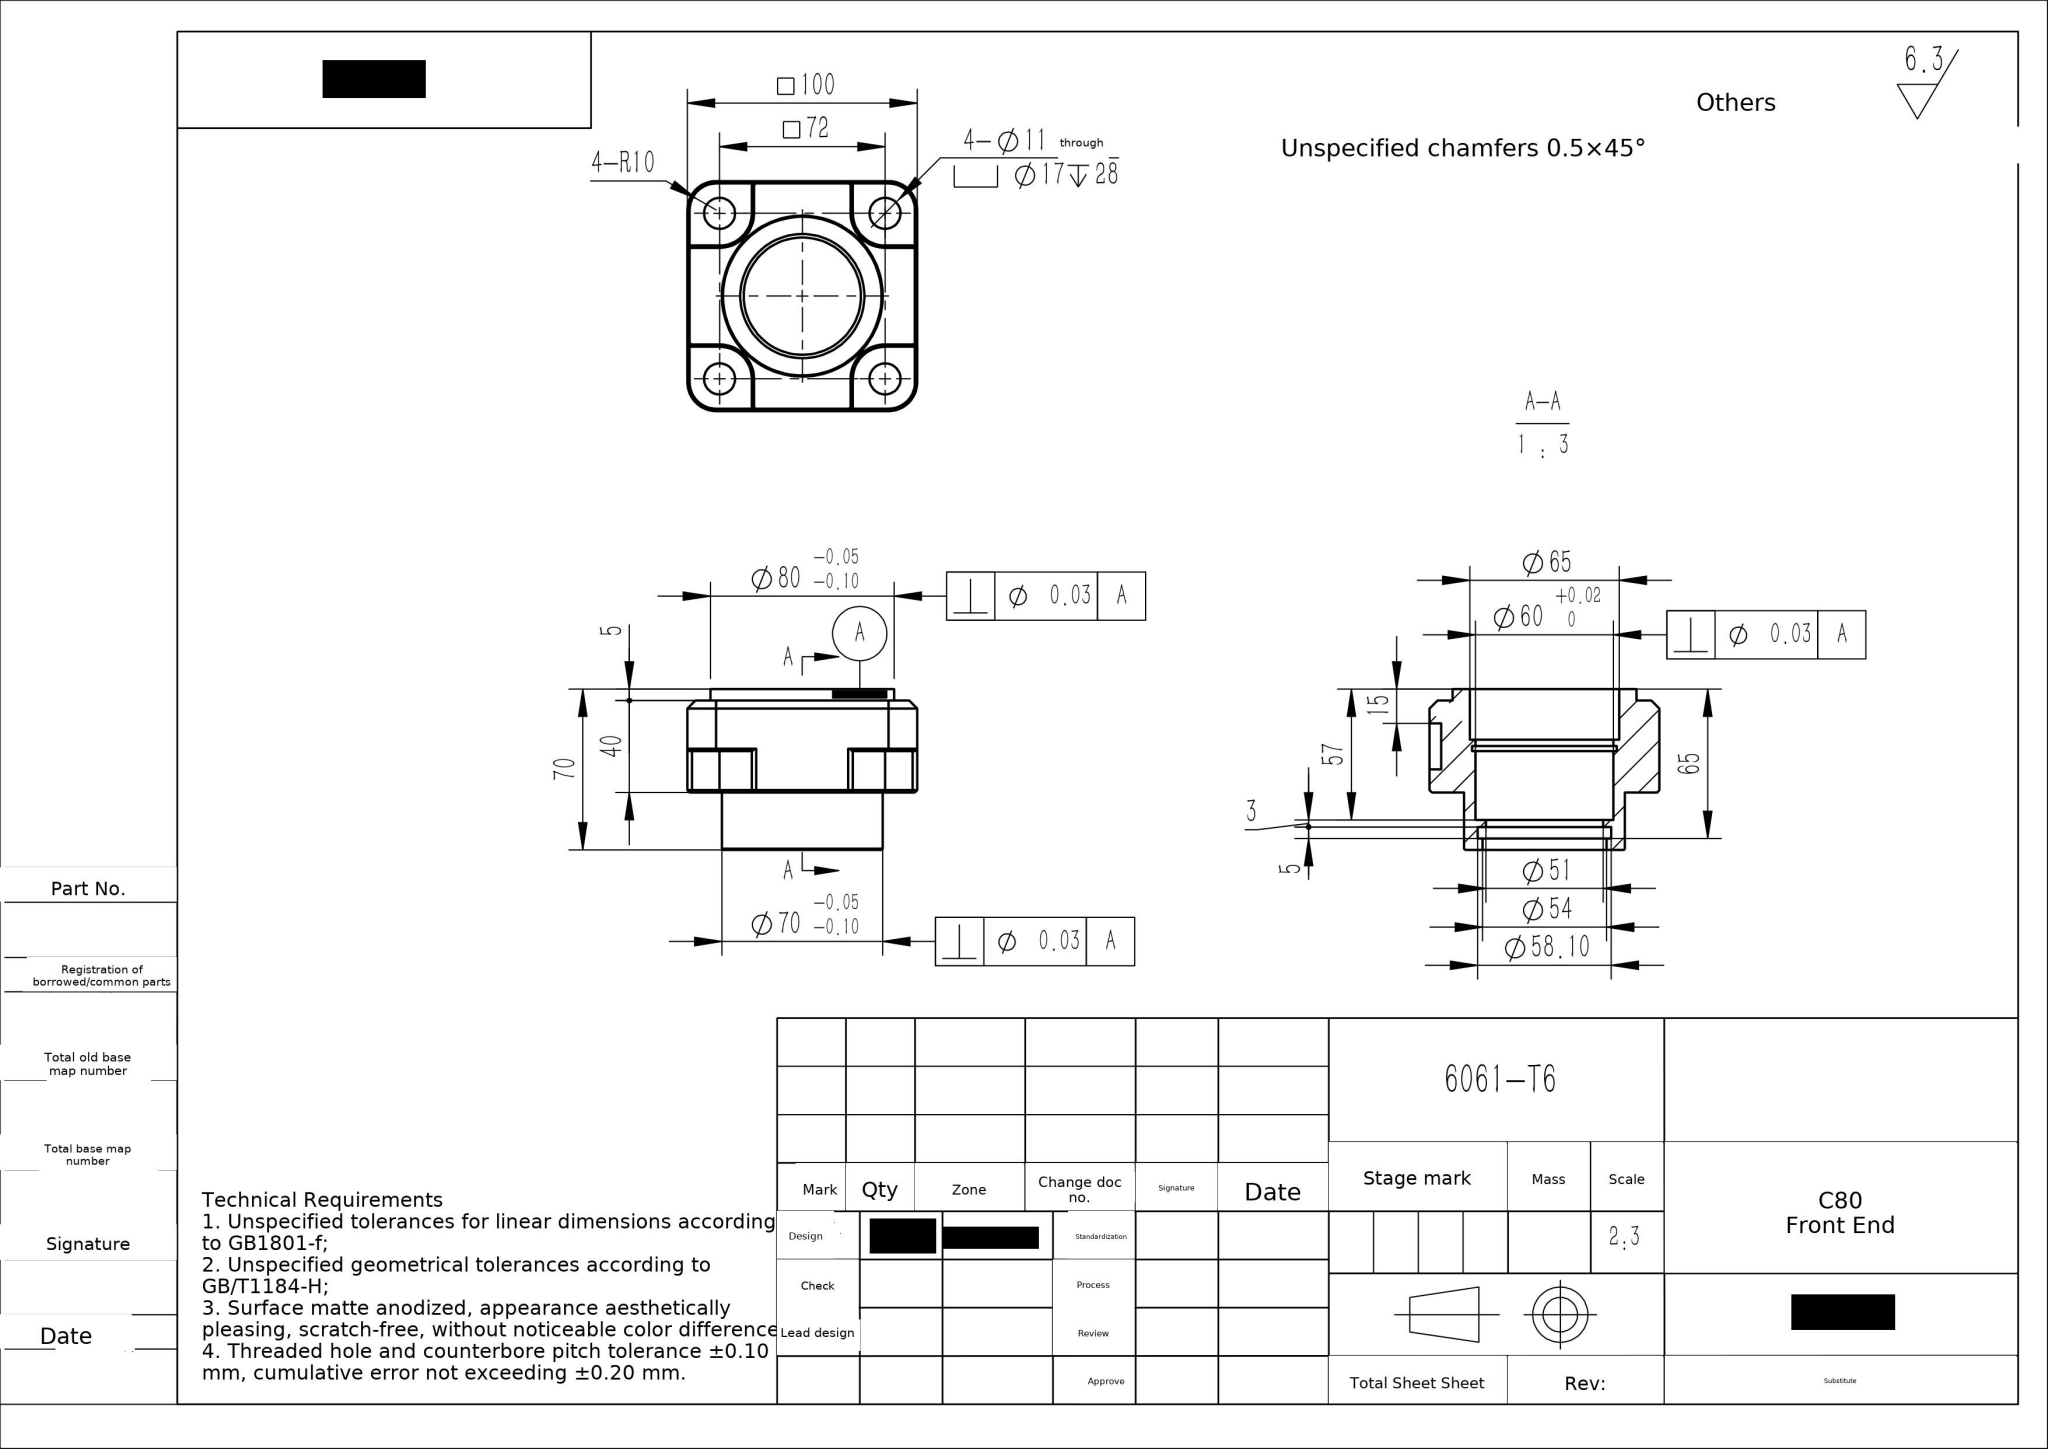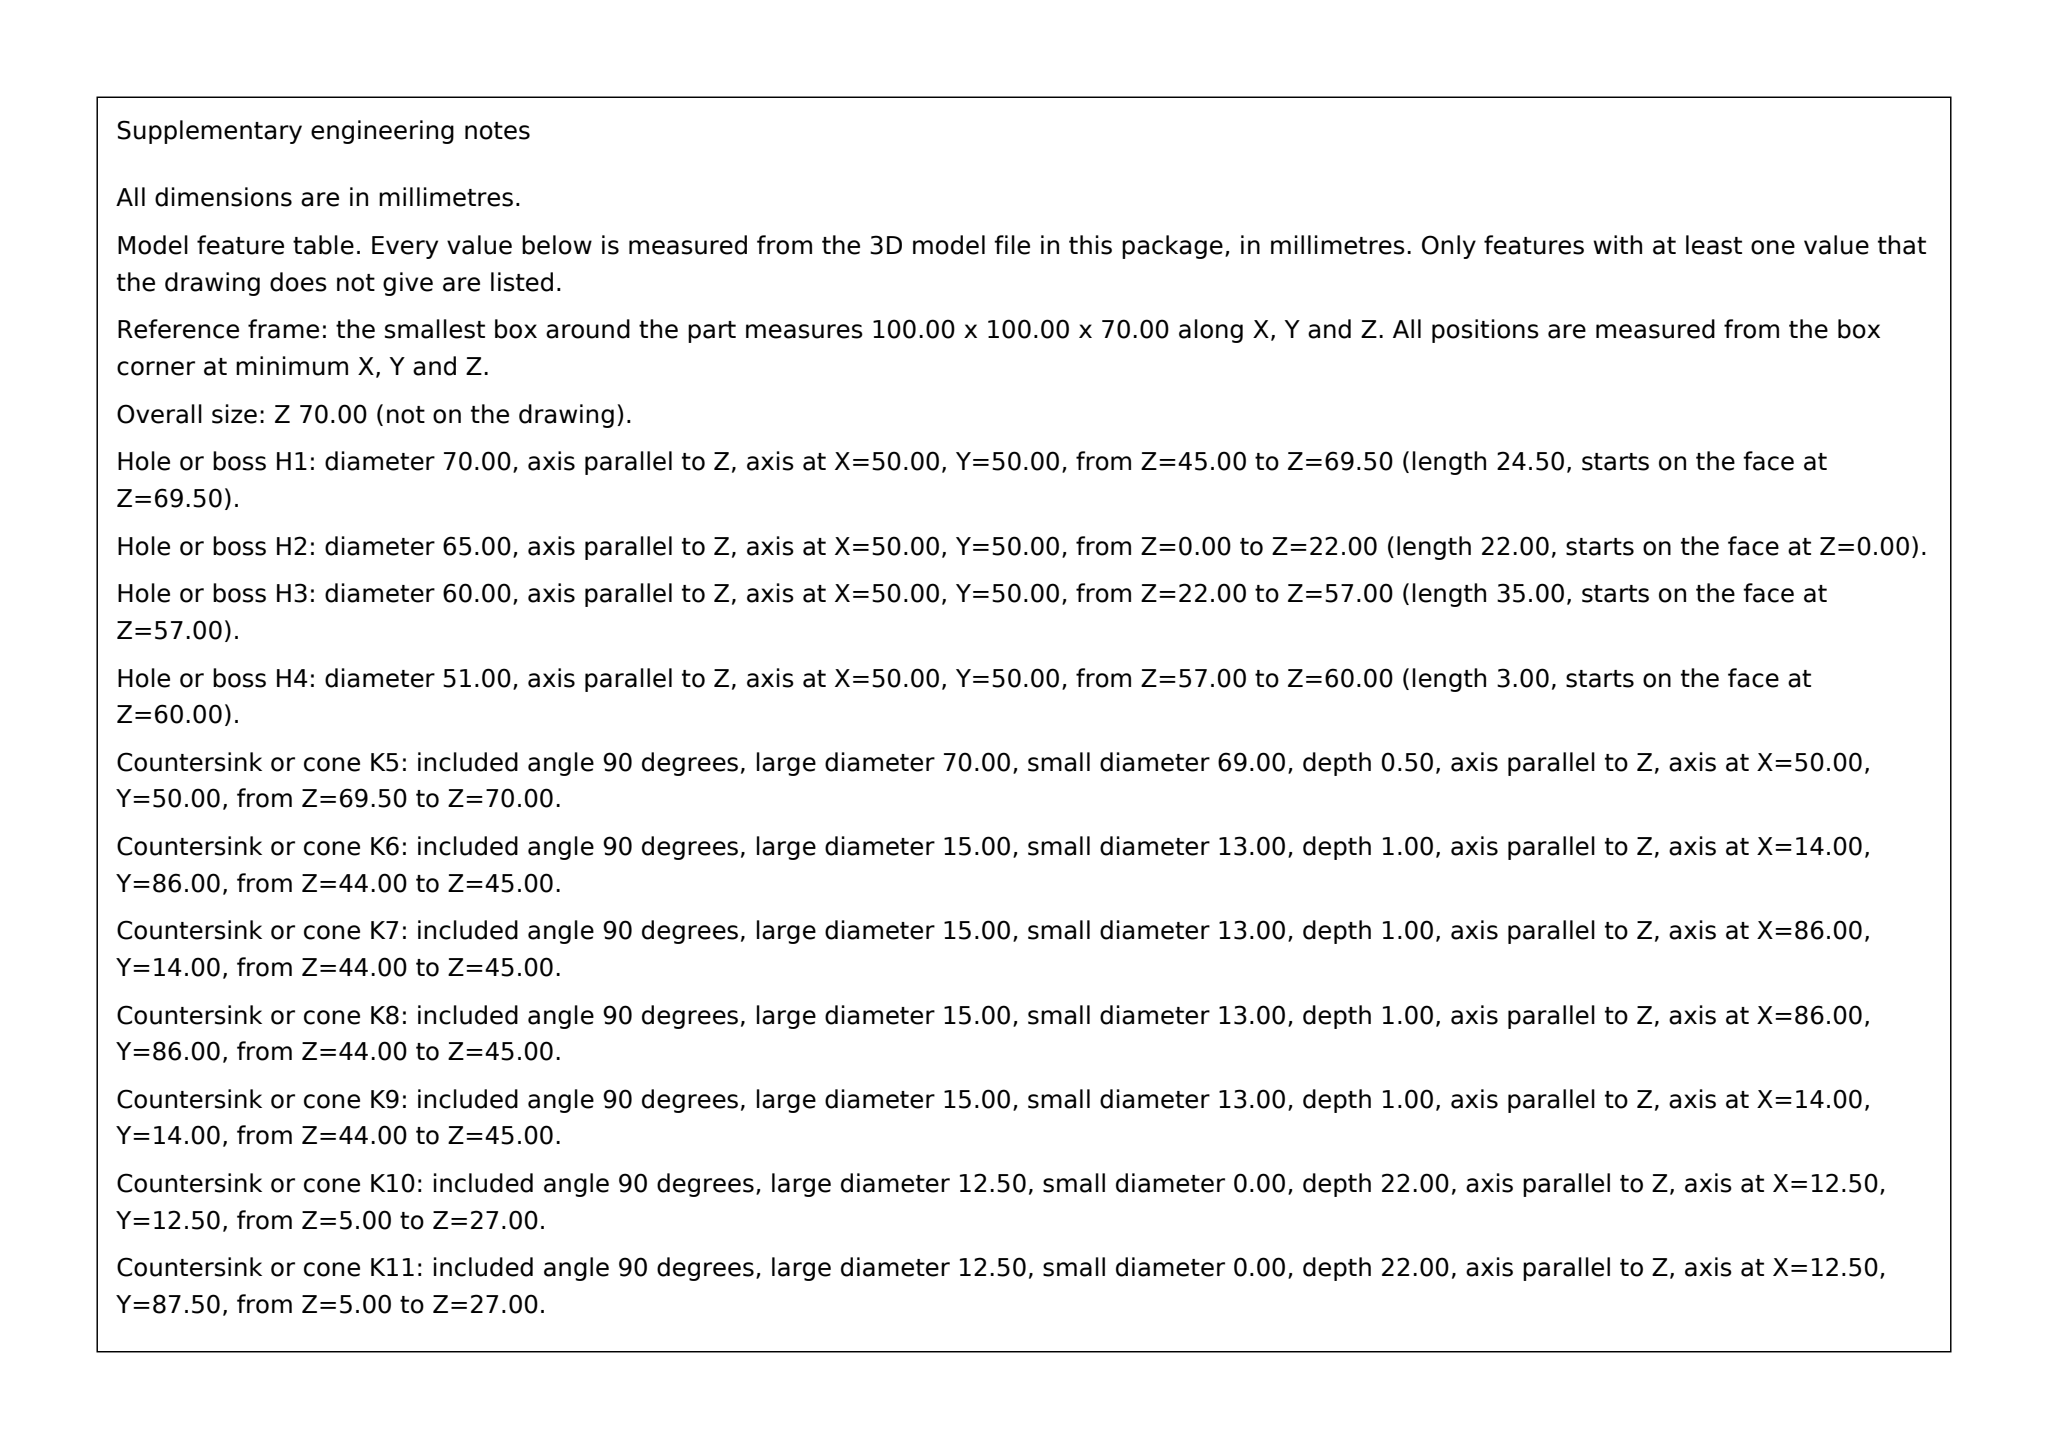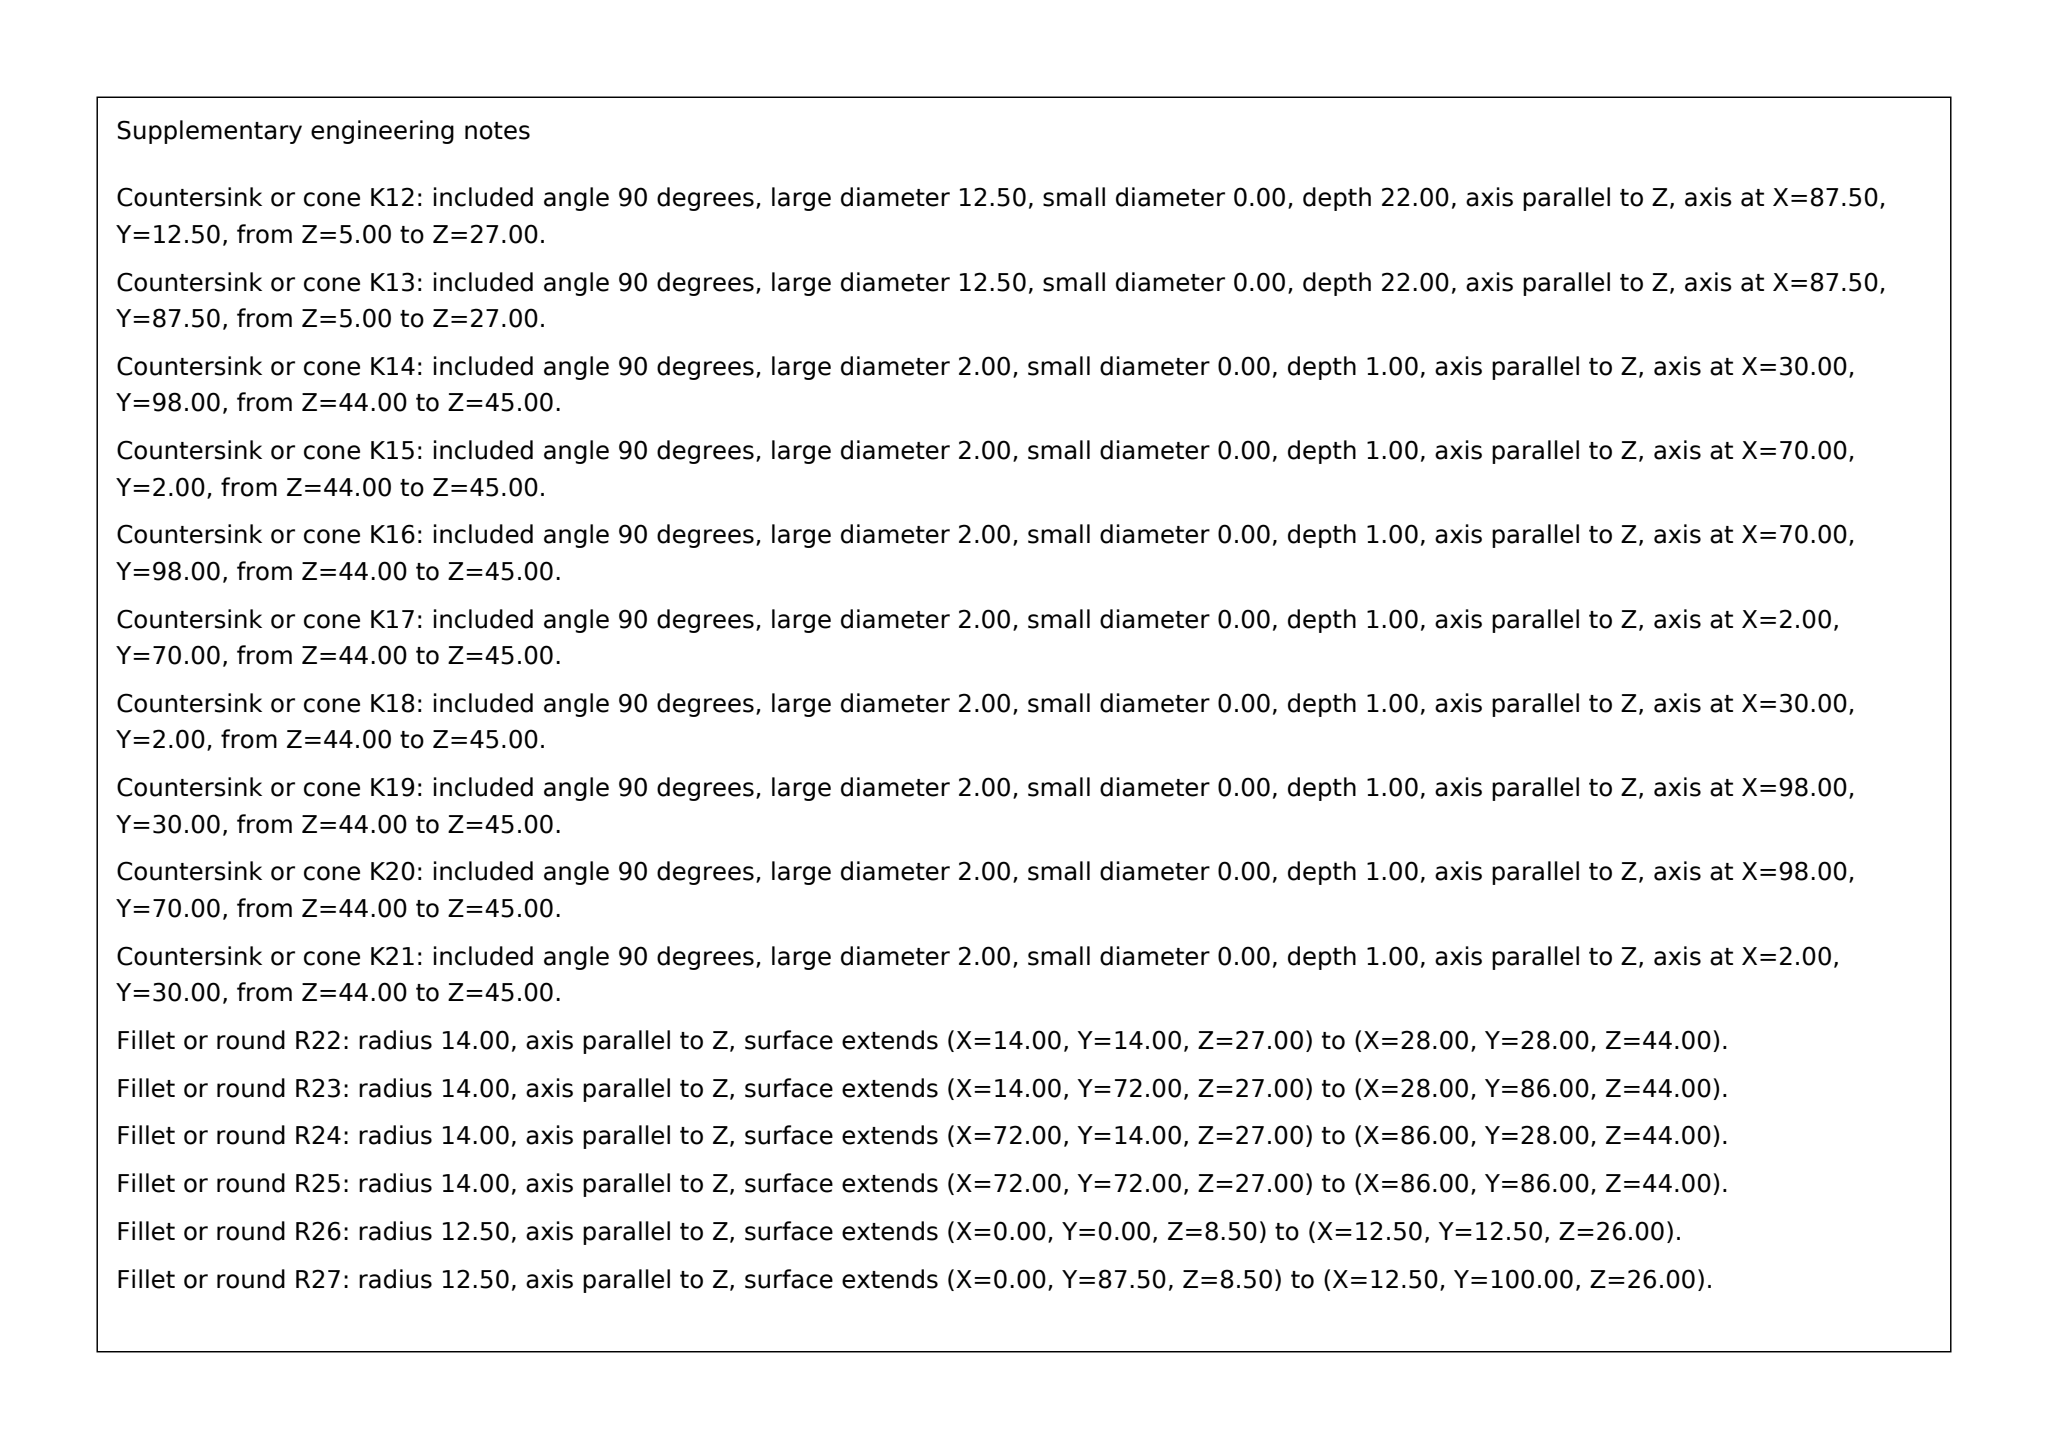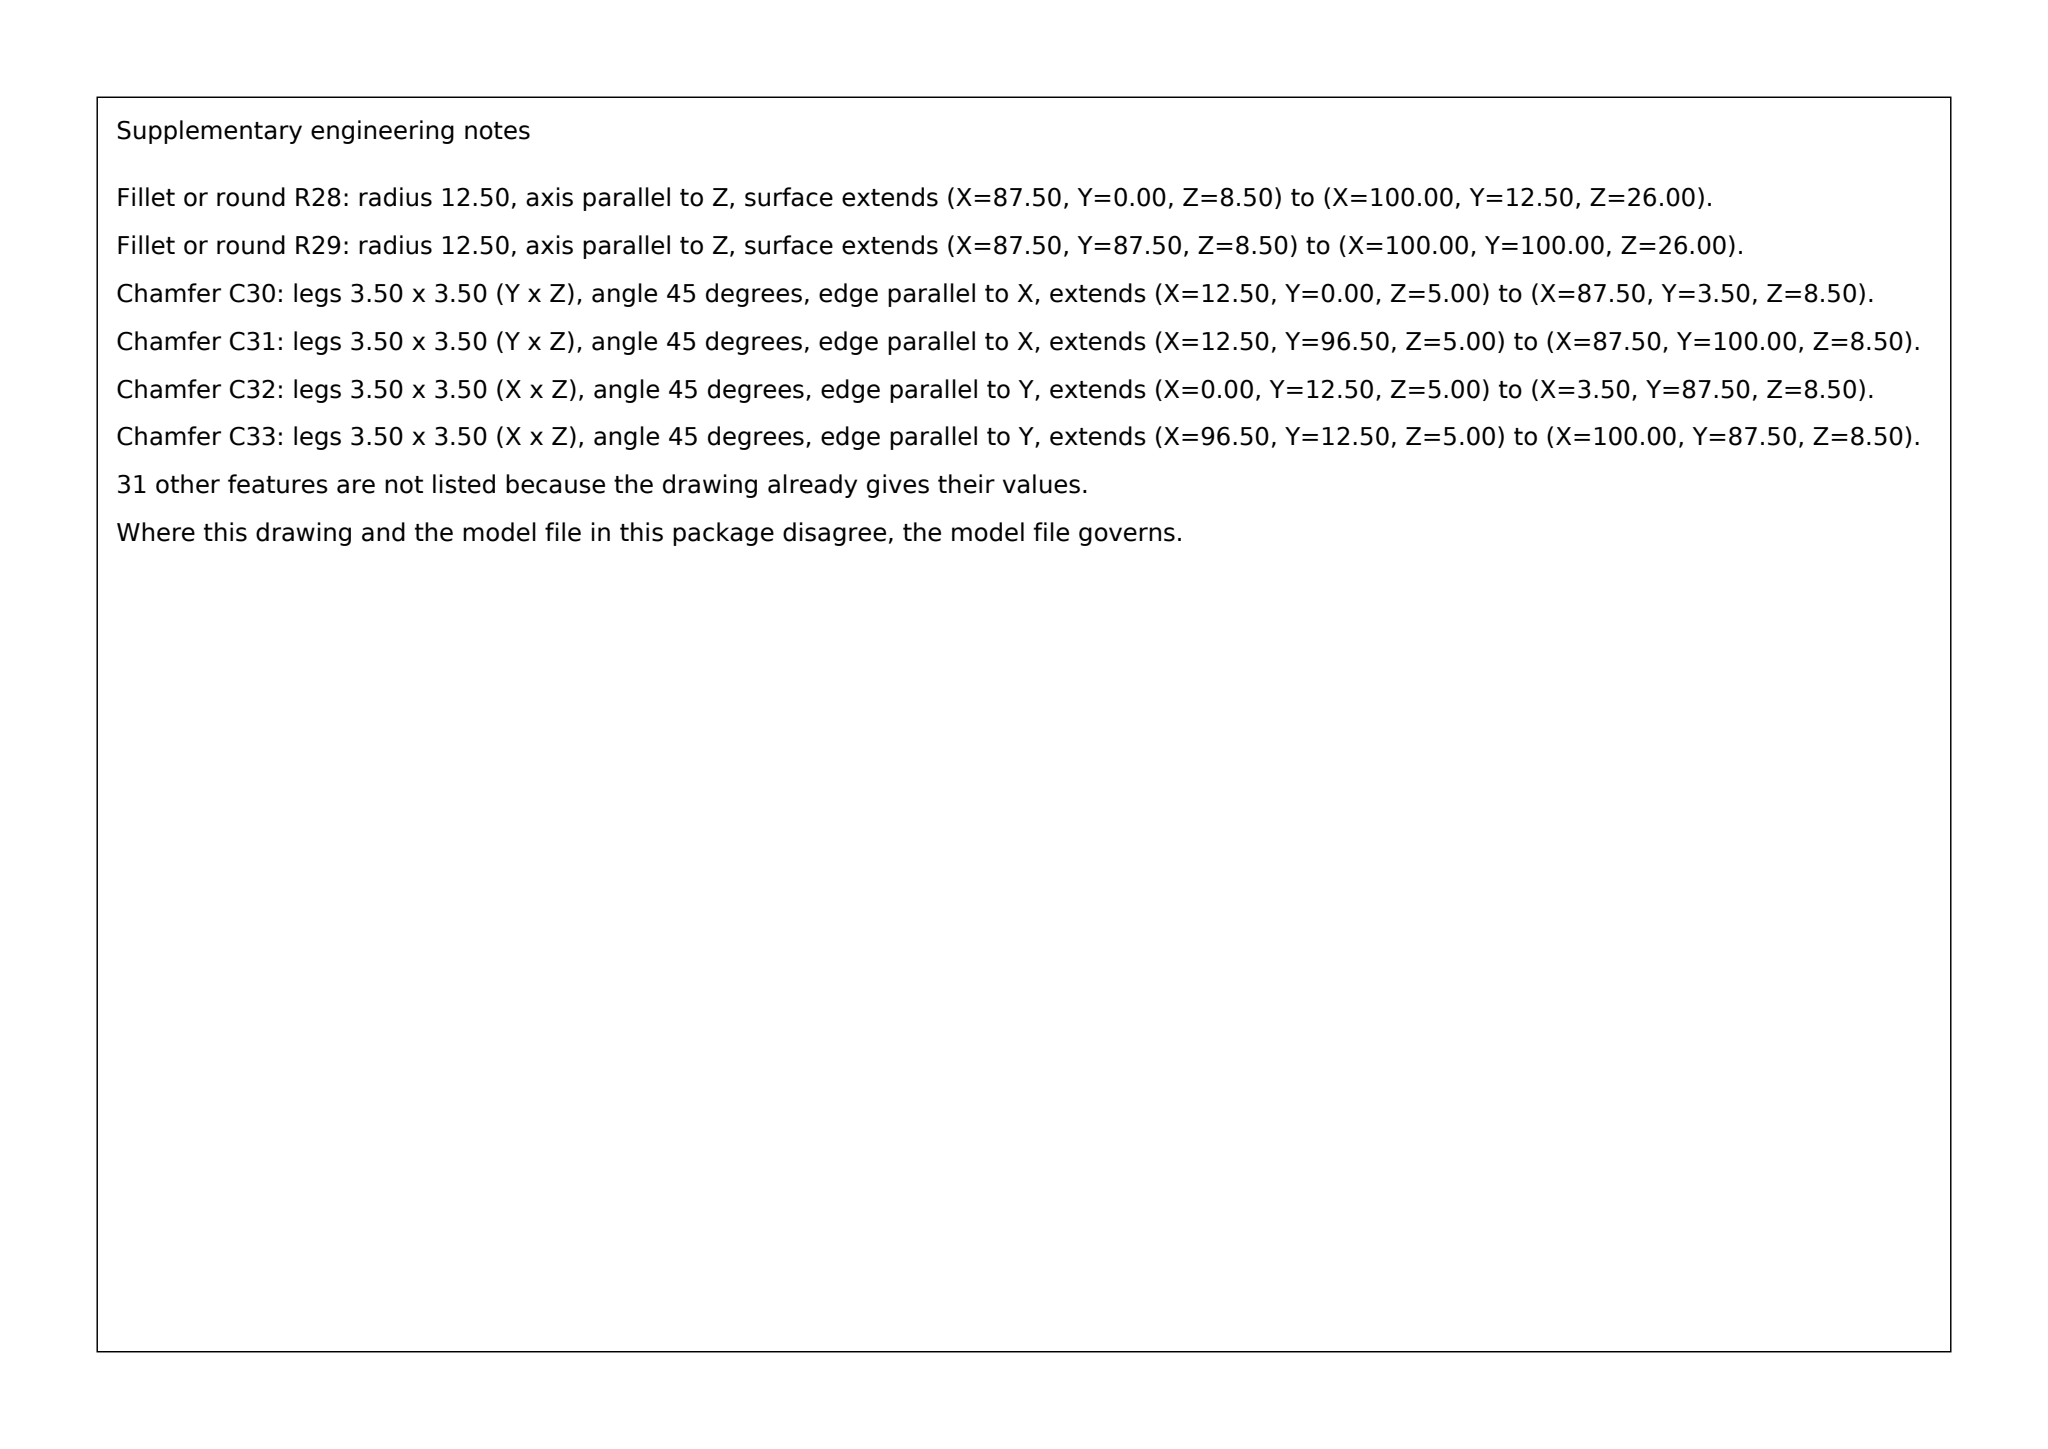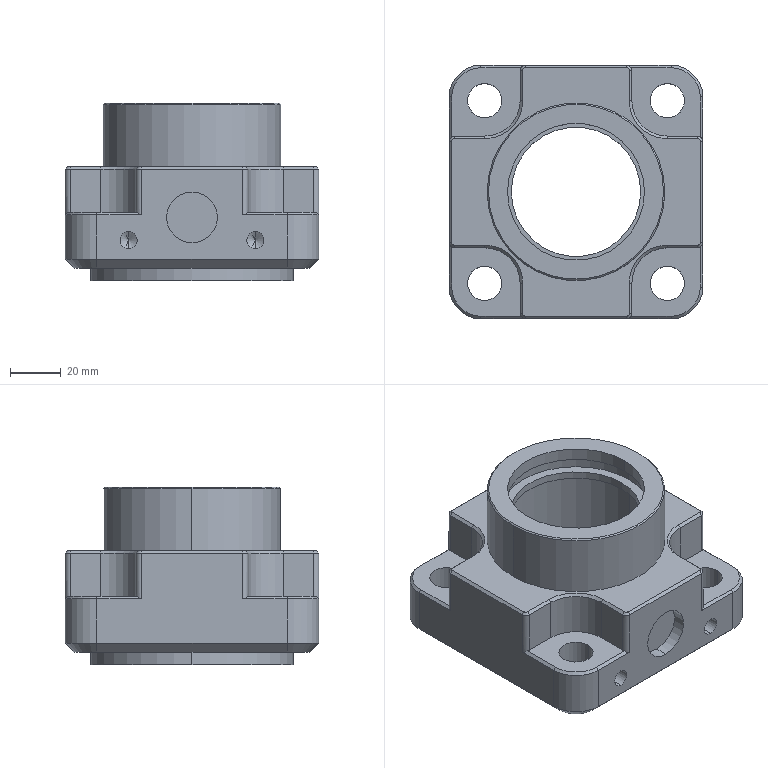Part | SolidWorks | mm | material 6061-T6 | 1 solid | 125 faces | box 100 x 100 x 70 mm | volume 243174 mm3 | plane 51 | cylinder 48 | cone 26 | commonest cylinder face diameters 13.5 x8 4 x8 6.8 x4 60 x4 25 x4 28 x4 20 x2 58.1 x2